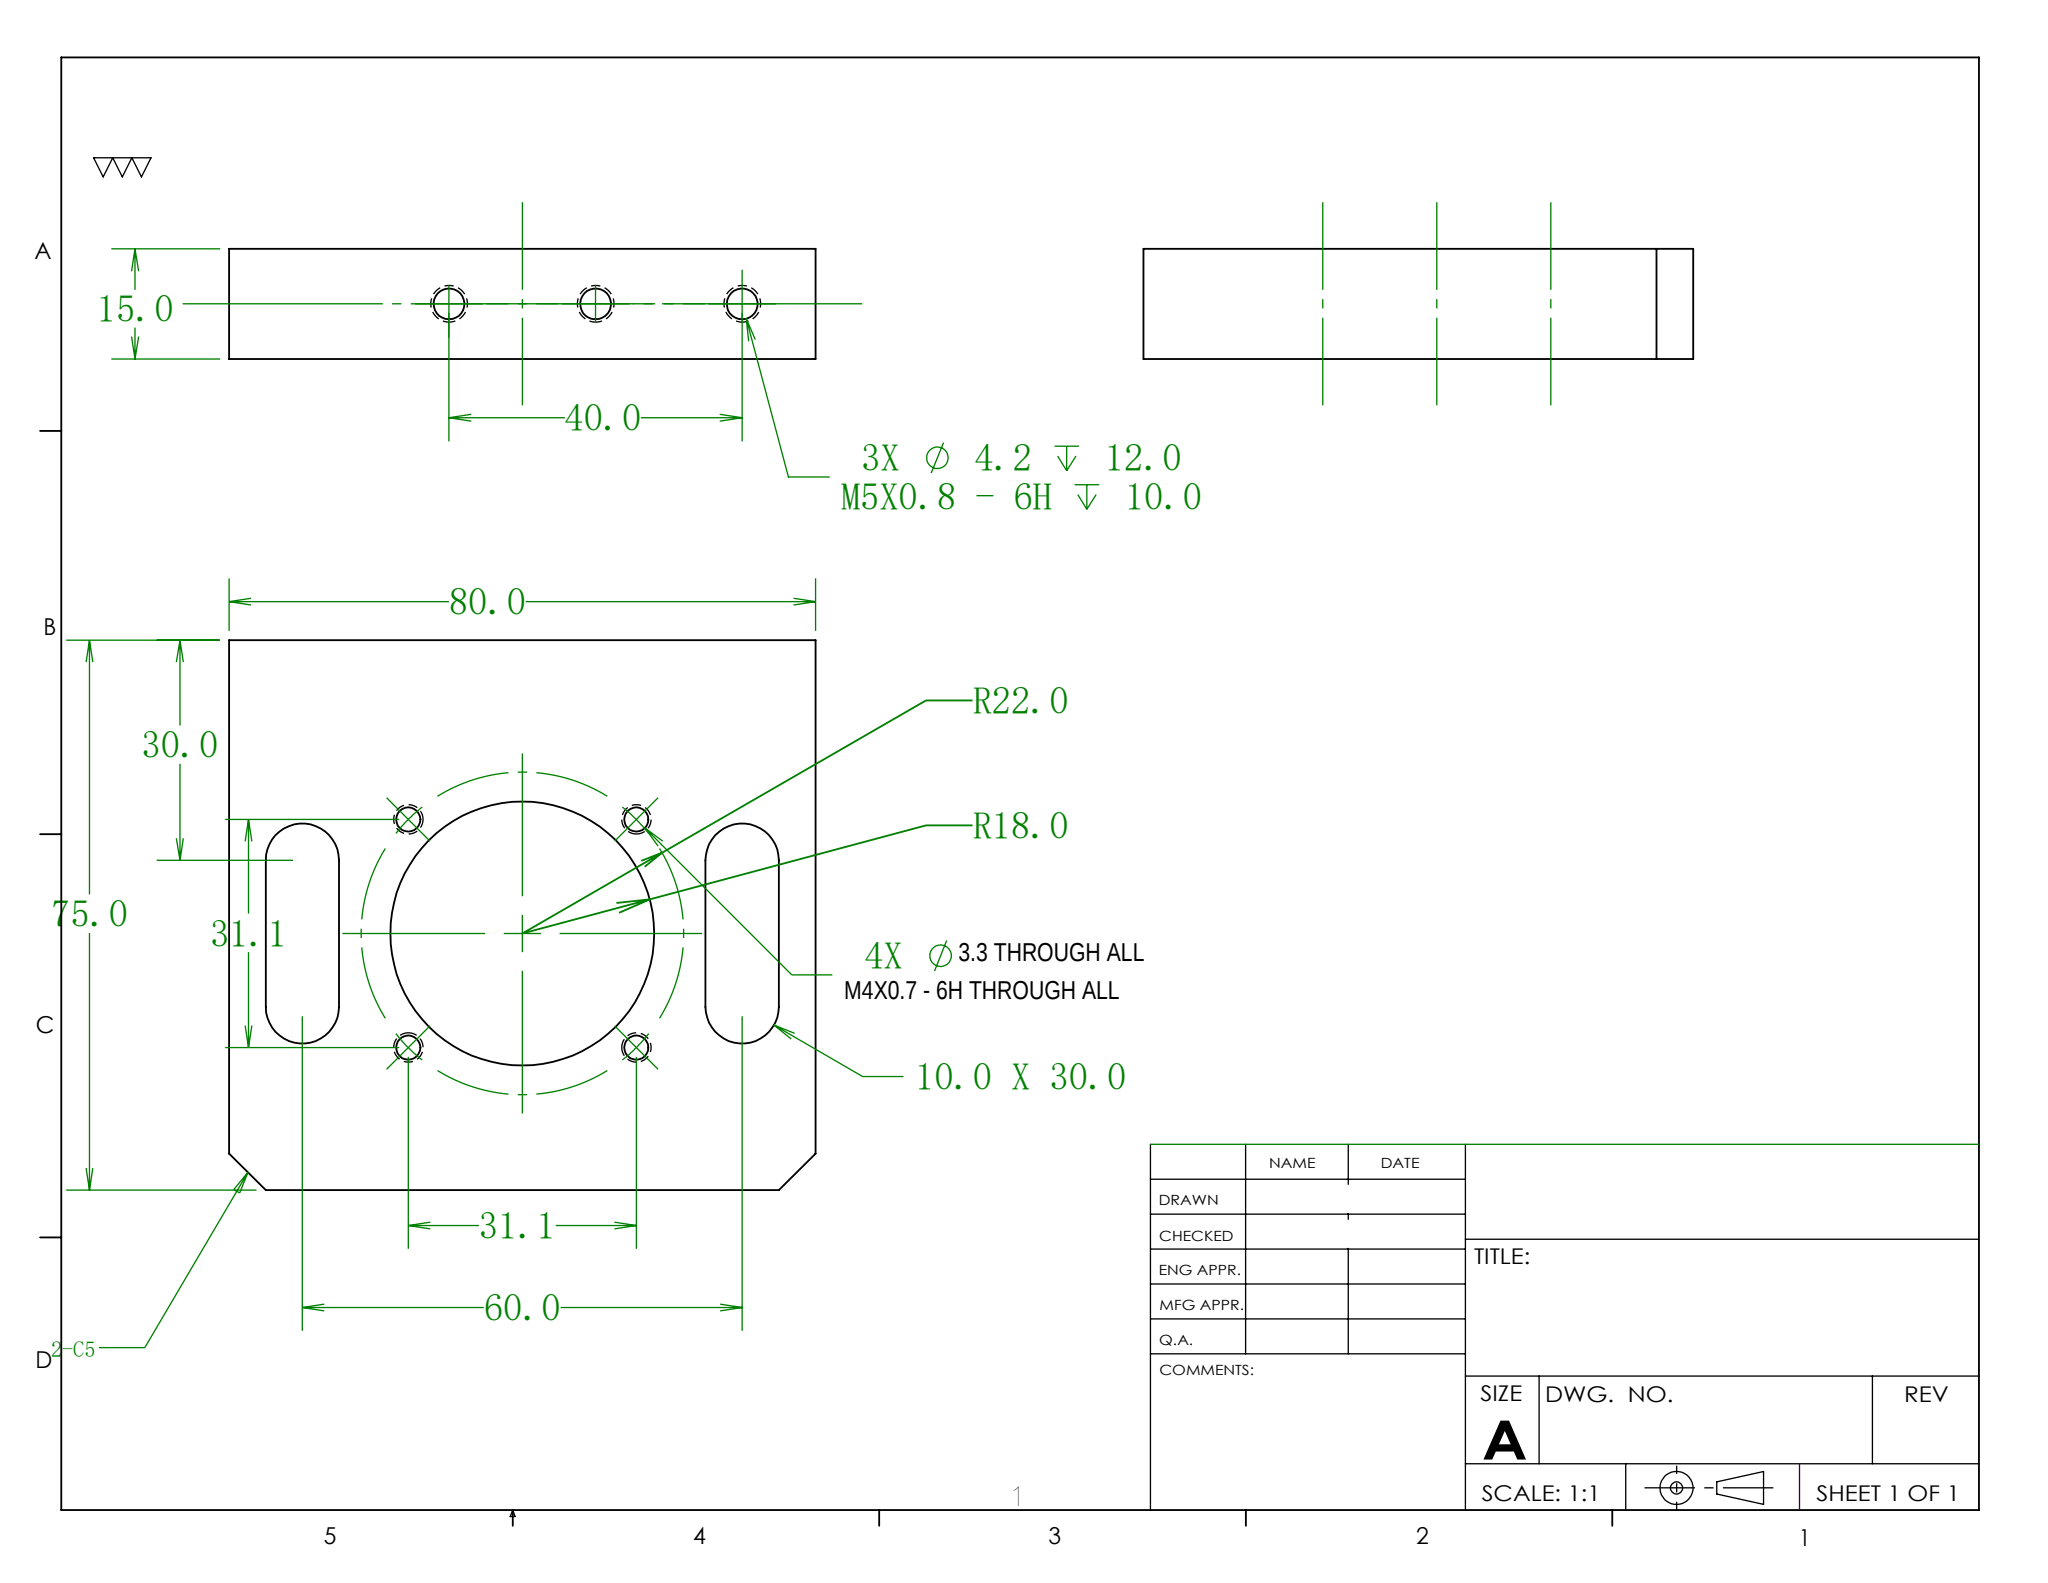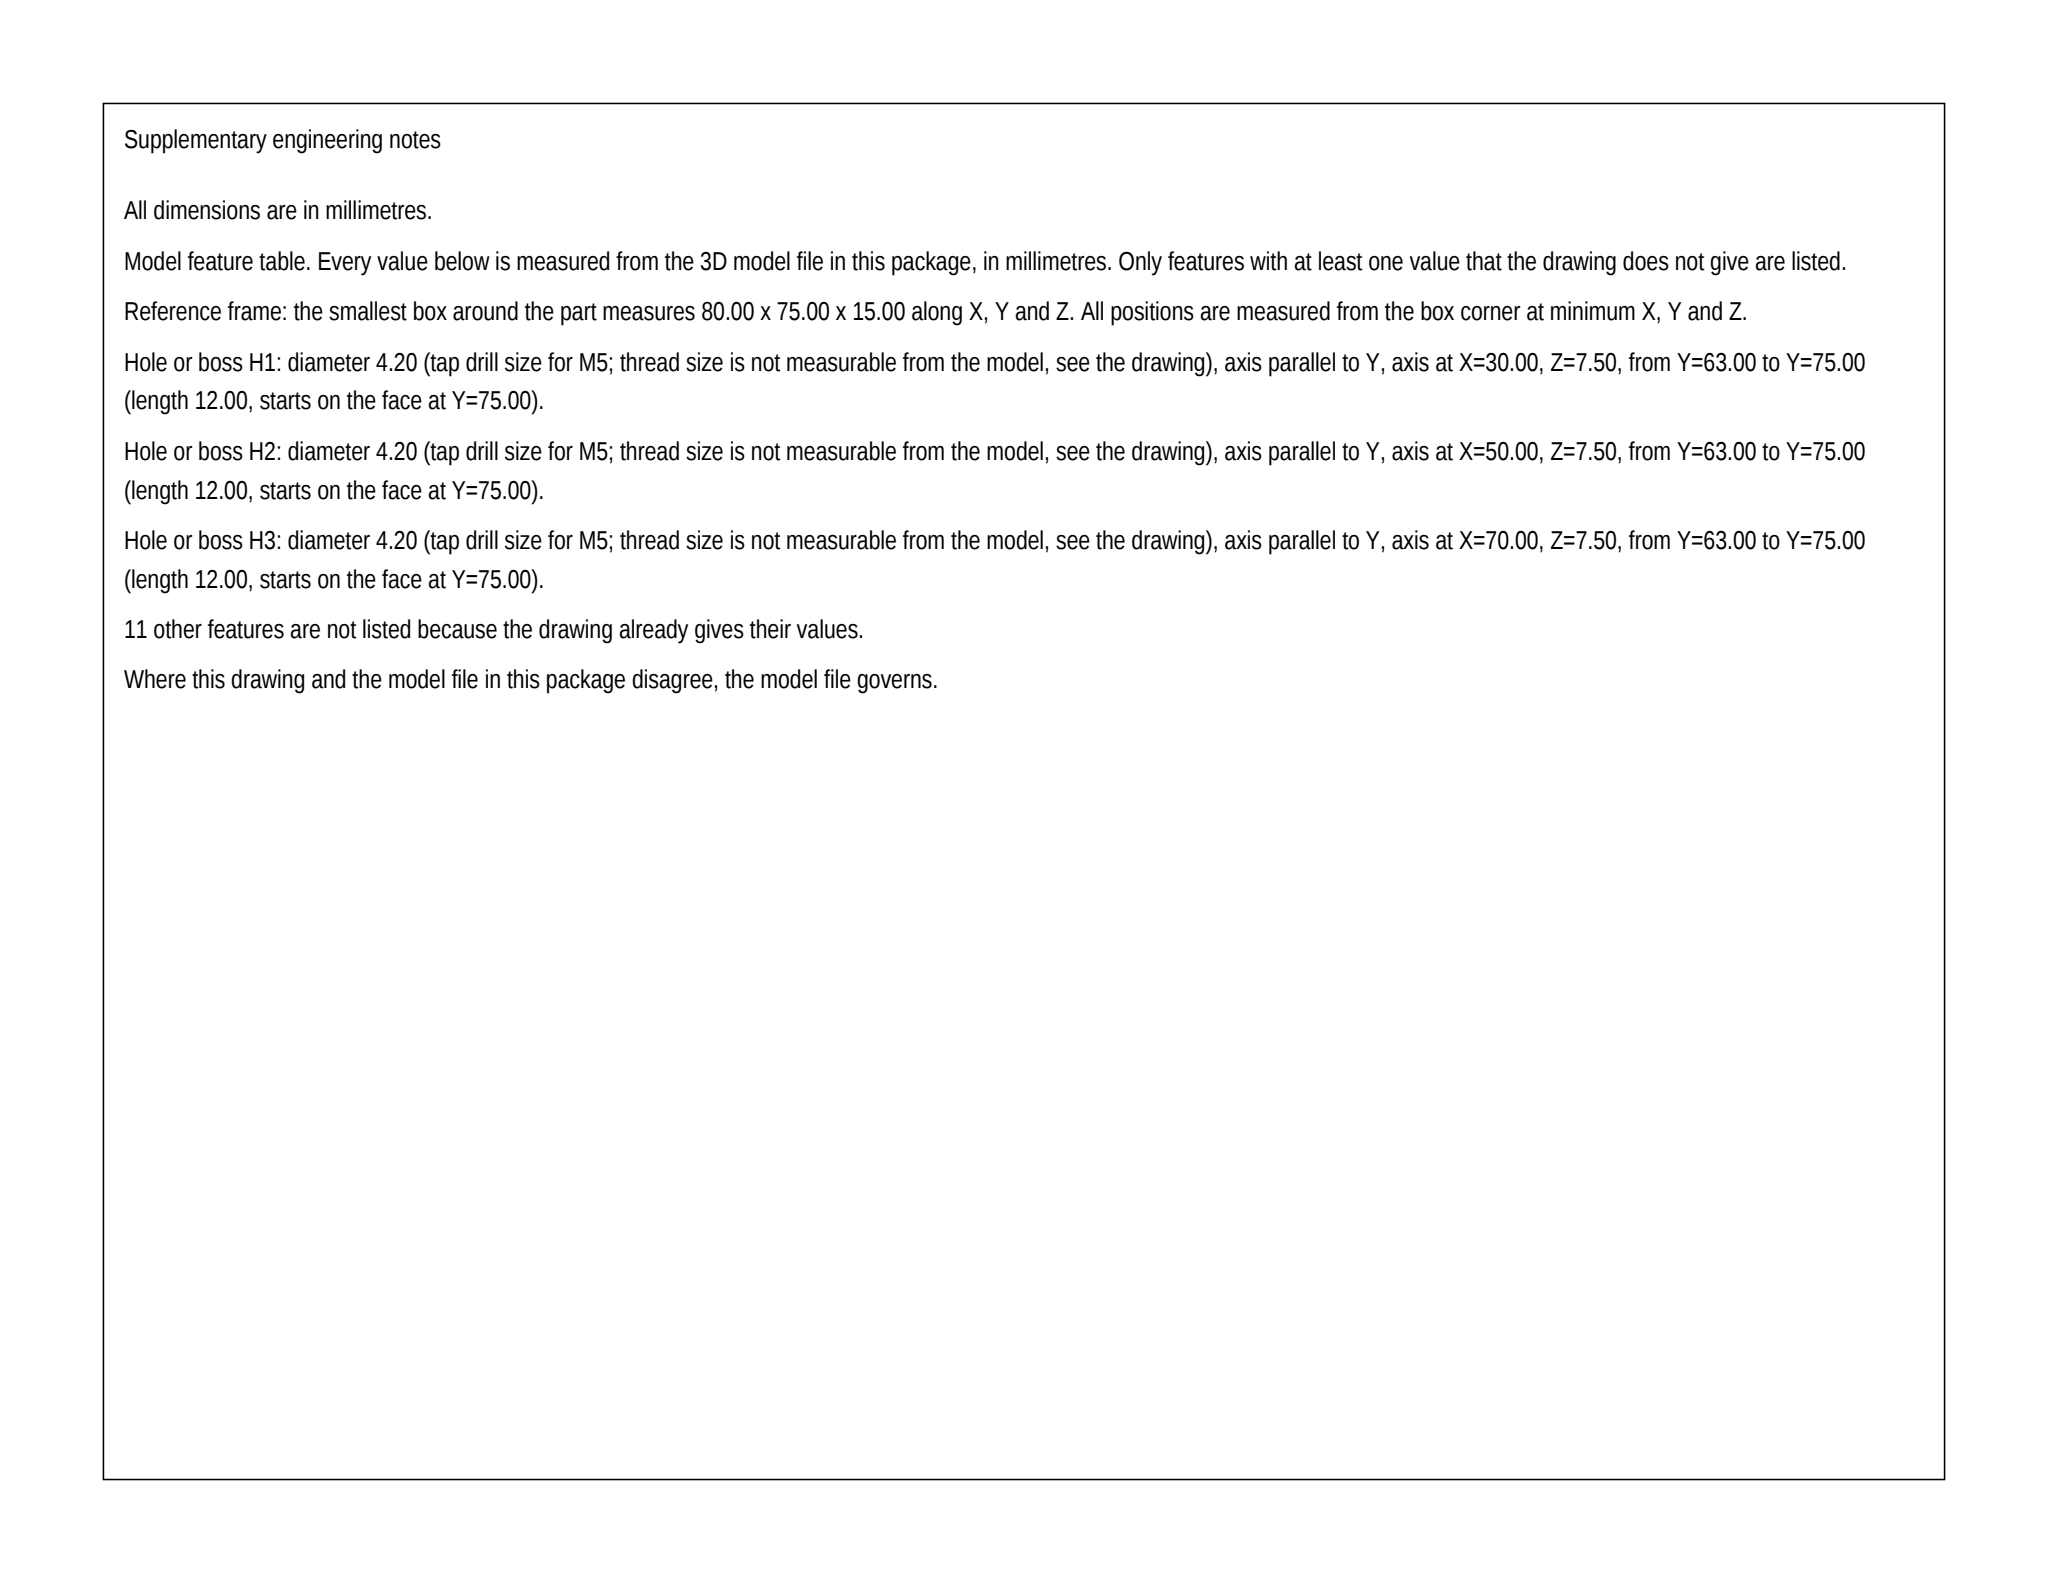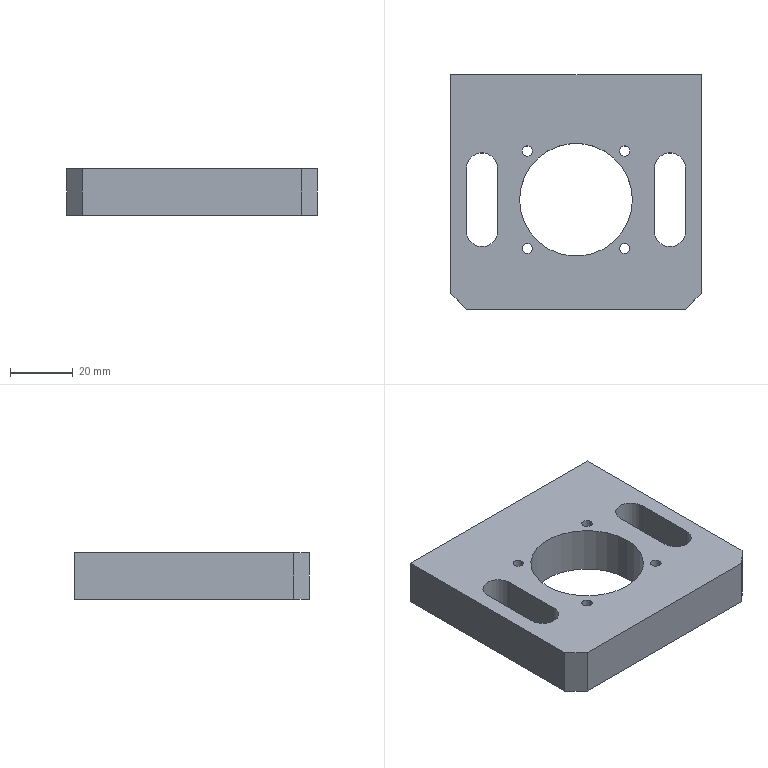Part | SolidWorks | mm | 1 solid | 38 faces | box 80 x 75 x 15 mm | volume 64971 mm3 | cylinder 20 | plane 12 | cone 6 | commonest cylinder face diameters 3.3 x8 4.2 x6 10 x4 36 x2
build123d program:
from build123d import *

# Parameters (mm, degrees)
SKETCH1_W             = 80
SKETCH1_H             = 80
EXTRUDE1_DEPTH        = 15
SKETCH2_R             = 18
CUT_EXTRUDE1_DEPTH    = 96.836
M4X0_7_TAPPED_HOLE1_D = 3.3
CIRPATTERN1_COUNT     = 4
LPATTERN1_COUNT       = 3
LPATTERN1_PITCH       = 20
SKETCH5_W             = 80
SKETCH5_H             = 5
CUT_EXTRUDE2_DEPTH    = 96.836
CHAMFER1_SIZE         = 5
CUT_EXTRUDE3_DEPTH    = 96.836


with BuildPart() as part:
    # Sketch1 → Extrude1 (new body)
    with BuildSketch(Plane.XY):
        with Locations((-32.259, 21.14)):
            Rectangle(SKETCH1_W, SKETCH1_H)
    extrude(amount=EXTRUDE1_DEPTH)

    # Sketch2 → Cut-Extrude1 (cut, through all)
    with BuildSketch(Plane.XY.offset(15)):
        with Locations((-32.259, 21.14)):
            Circle(SKETCH2_R)
    extrude(amount=-CUT_EXTRUDE1_DEPTH, mode=Mode.SUBTRACT)

    # M4x0.7 Tapped Hole1 (through all)
    with Locations(Plane(origin=(-16.703, 36.696, 15), x_dir=(1, 0, 0), z_dir=(0, 0, 1))):
        with Locations((0, 0)):
            m4x0_7_tapped_hole1 = Hole(M4X0_7_TAPPED_HOLE1_D / 2)

    # CirPattern1: M4x0.7 Tapped Hole1 ×4 about axis
    cirpattern1_axis = Axis((-32.259, 21.14, 0), (0, 0, 1))
    for i in range(1, CIRPATTERN1_COUNT):
        add(m4x0_7_tapped_hole1.rotate(cirpattern1_axis, i * 360 / CIRPATTERN1_COUNT), mode=Mode.SUBTRACT)

    # Sketch4 → M5x0.8 Tapped Hole1 (revolve, cut)
    with BuildSketch(Plane(origin=(-2.259, 61.14, 7.5), x_dir=(0, 0, 1), z_dir=(1, 0, 0))):
        Polygon((0, 0), (0, 13.262), (2.1, 12), (2.1, 0), align=None)
    m5x0_8_tapped_hole1 = revolve(axis=Axis((-2.259, 67.49, 7.5), (0, -1, 0)), mode=Mode.SUBTRACT)

    # LPattern1: M5x0.8 Tapped Hole1 ×3
    with Locations(*[(-i * LPATTERN1_PITCH, 0, 0) for i in range(1, LPATTERN1_COUNT)]):
        add(m5x0_8_tapped_hole1, mode=Mode.SUBTRACT)

    # Sketch5 → Cut-Extrude2 (cut, through all)
    with BuildSketch(Plane(origin=(0, 0, 0), x_dir=(-1, 0, 0), z_dir=(0, 0, -1))):
        with Locations((32.259, -16.36)):
            Rectangle(SKETCH5_W, SKETCH5_H)
    extrude(amount=-CUT_EXTRUDE2_DEPTH, mode=Mode.SUBTRACT)

    # Chamfer1
    chamfer1_edges = [part.edges().sort_by_distance(p)[0] for p in [
        (7.741, -13.86, 7.5),
        (-72.259, -13.86, 7.5),
    ]]
    chamfer(chamfer1_edges, length=CHAMFER1_SIZE)

    # Sketch6 → Cut-Extrude3 (cut, through all)
    with BuildSketch(Plane(origin=(0, 0, 0), x_dir=(-1, 0, 0), z_dir=(0, 0, -1))):
        with BuildLine():
            Line((7.259, 31.14), (7.259, 11.14))
            ThreePointArc((7.259, 11.14), (2.259, 6.14), (-2.741, 11.14))
            Line((-2.741, 11.14), (-2.741, 31.14))
            ThreePointArc((-2.741, 31.14), (2.259, 36.14), (7.259, 31.14))
        make_face()
        with BuildLine():
            Line((67.259, 31.14), (67.259, 11.14))
            ThreePointArc((67.259, 11.14), (62.259, 6.14), (57.259, 11.14))
            Line((57.259, 11.14), (57.259, 31.14))
            ThreePointArc((57.259, 31.14), (62.259, 36.14), (67.259, 31.14))
        make_face()
    extrude(amount=-CUT_EXTRUDE3_DEPTH, mode=Mode.SUBTRACT)


solid = part.part